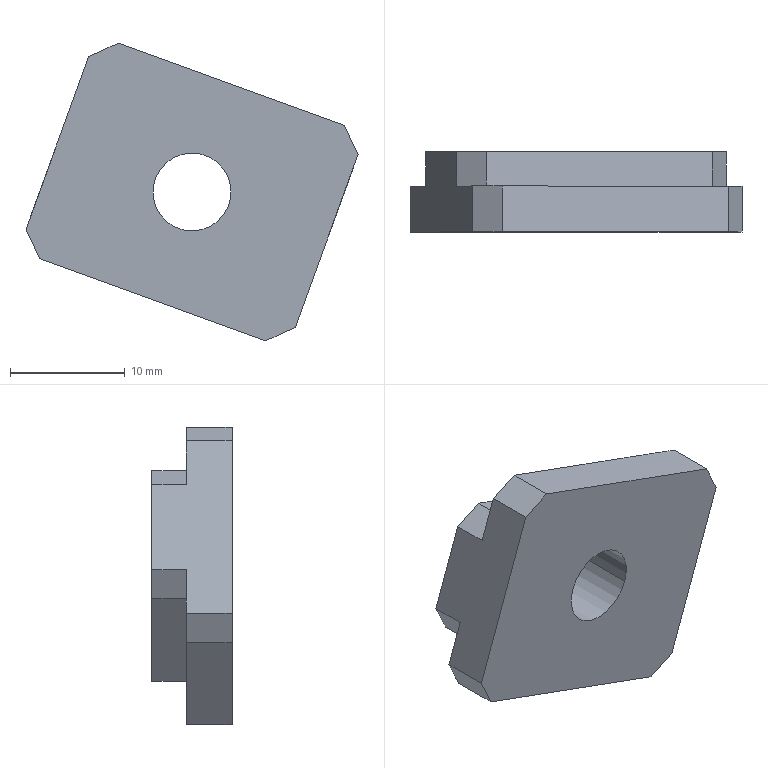Component | SolidWorks | MA060.03.03-07-10 | 1 solid | 20 faces | box 28.96 x 7 x 25.98 mm | volume 2582 mm3 | plane 18 | cylinder 2 | commonest cylinder face diameters 6.8 x2 | material Q235A
build123d program:
from build123d import *

# Parameters (mm, degrees)
SKETCH1_W           = 25
SKETCH1_H           = 20
BOSS_EXTRUDE1_DEPTH = 7
M8_TAPPED_HOLE1_D   = 6.8
SKETCH4_W           = 3
SKETCH4_H           = 4.05
CUT_EXTRUDE1_DEPTH  = 28.821
CHAMFER1_SIZE       = 2


with BuildPart() as part:
    # Sketch1 → Boss-Extrude1 (new body)
    with BuildSketch(Plane.XY):
        Rectangle(SKETCH1_W, SKETCH1_H)
    extrude(amount=BOSS_EXTRUDE1_DEPTH)

    # M8 Tapped Hole1 (through all)
    with Locations(Plane.XY.offset(7)):
        with Locations((0, 0)):
            Hole(M8_TAPPED_HOLE1_D / 2)

    # Sketch4 → Cut-Extrude1 (cut, through all)
    with BuildSketch(Plane(origin=(12.5, 0, 0), x_dir=(0, 0, -1), z_dir=(1, 0, 0))):
        with Locations((-1.5, 7.975)):
            Rectangle(SKETCH4_W, SKETCH4_H)
        with Locations((-1.5, -7.975)):
            Rectangle(SKETCH4_W, SKETCH4_H)
    extrude(amount=-CUT_EXTRUDE1_DEPTH, mode=Mode.SUBTRACT)

    # Chamfer1
    chamfer1_edges = [part.edges().sort_by_distance(p)[0] for p in [
        (-12.5, 5.95, 1.5),
        (12.5, 5.95, 1.5),
        (-12.5, -5.95, 1.5),
        (12.5, -5.95, 1.5),
        (12.5, -10, 5),
        (-12.5, -10, 5),
        (-12.5, 10, 5),
        (12.5, 10, 5),
    ]]
    chamfer(chamfer1_edges, length=CHAMFER1_SIZE)


solid = part.part

# Placed as in the assembly
solid = solid.moved(Location((221.425, 81.053, -80.645), (90, 0, -20)))
STEP:
#1=COLOUR_RGB('',0.7922,0.8196,0.9333);
#2=FILL_AREA_STYLE_COLOUR('',#1);
#3=FILL_AREA_STYLE('',(#2));
#4=SURFACE_STYLE_FILL_AREA(#3);
#5=SURFACE_SIDE_STYLE('',(#4));
#6=SURFACE_STYLE_USAGE(.BOTH.,#5);
#7=PRESENTATION_STYLE_ASSIGNMENT((#6));
#8=CARTESIAN_POINT('',(8.843,3.191,-3.221));
#9=VERTEX_POINT('',#8);
#10=CARTESIAN_POINT('',(8.592,3.191,-3.129));
#11=VERTEX_POINT('',#10);
#12=CARTESIAN_POINT('',(8.718,3.191,-3.175));
#13=DIRECTION('',(-0.,-1.,0.));
#14=DIRECTION('',(-0.9397,0.,0.342));
#15=AXIS2_PLACEMENT_3D('',#12,#13,#14);
#16=CIRCLE('',#15,0.1339);
#17=EDGE_CURVE('',#9,#11,#16,.T.);
#18=ORIENTED_EDGE('',*,*,#17,.F.);
#19=CARTESIAN_POINT('',(8.843,2.915,-3.221));
#20=VERTEX_POINT('',#19);
#21=CARTESIAN_POINT('',(8.843,2.915,-3.221));
#22=DIRECTION('',(-0.,-1.,0.));
#23=VECTOR('',#22,39.37);
#24=LINE('',#21,#23);
#25=EDGE_CURVE('',#9,#20,#24,.T.);
#26=ORIENTED_EDGE('',*,*,#25,.T.);
#27=CARTESIAN_POINT('',(8.592,2.915,-3.129));
#28=VERTEX_POINT('',#27);
#29=CARTESIAN_POINT('',(8.718,2.915,-3.175));
#30=DIRECTION('',(-0.,-1.,0.));
#31=DIRECTION('',(-0.9397,0.,0.342));
#32=AXIS2_PLACEMENT_3D('',#29,#30,#31);
#33=CIRCLE('',#32,0.1339);
#34=EDGE_CURVE('',#20,#28,#33,.T.);
#35=ORIENTED_EDGE('',*,*,#34,.T.);
#36=CARTESIAN_POINT('',(8.592,2.915,-3.129));
#37=DIRECTION('',(-0.,-1.,0.));
#38=VECTOR('',#37,39.37);
#39=LINE('',#36,#38);
#40=EDGE_CURVE('',#11,#28,#39,.T.);
#41=ORIENTED_EDGE('',*,*,#40,.F.);
#42=EDGE_LOOP('',(#18,#26,#35,#41));
#43=FACE_OUTER_BOUND('',#42,.T.);
#44=CARTESIAN_POINT('',(8.718,2.915,-3.175));
#45=DIRECTION('',(-0.,-1.,0.));
#46=DIRECTION('',(-0.9397,0.,0.342));
#47=AXIS2_PLACEMENT_3D('',#44,#45,#46);
#48=CYLINDRICAL_SURFACE('',#47,0.1339);
#49=ADVANCED_FACE('',(#43),#48,.F.);
#50=CARTESIAN_POINT('',(8.308,3.073,-2.861));
#51=VERTEX_POINT('',#50);
#52=CARTESIAN_POINT('',(8.363,3.073,-2.711));
#53=VERTEX_POINT('',#52);
#54=CARTESIAN_POINT('',(8.39,3.073,-2.637));
#55=DIRECTION('',(0.342,-0.,0.9397));
#56=VECTOR('',#55,39.37);
#57=LINE('',#54,#56);
#58=EDGE_CURVE('',#51,#53,#57,.T.);
#59=ORIENTED_EDGE('',*,*,#58,.F.);
#60=CARTESIAN_POINT('',(8.308,3.191,-2.861));
#61=VERTEX_POINT('',#60);
#62=CARTESIAN_POINT('',(8.308,2.915,-2.861));
#63=DIRECTION('',(0.,1.,-0.));
#64=VECTOR('',#63,39.37);
#65=LINE('',#62,#64);
#66=EDGE_CURVE('',#51,#61,#65,.T.);
#67=ORIENTED_EDGE('',*,*,#66,.T.);
#68=CARTESIAN_POINT('',(8.202,3.191,-3.153));
#69=VERTEX_POINT('',#68);
#70=CARTESIAN_POINT('',(8.39,3.191,-2.637));
#71=DIRECTION('',(-0.342,0.,-0.9397));
#72=VECTOR('',#71,39.37);
#73=LINE('',#70,#72);
#74=EDGE_CURVE('',#61,#69,#73,.T.);
#75=ORIENTED_EDGE('',*,*,#74,.T.);
#76=CARTESIAN_POINT('',(8.202,3.073,-3.153));
#77=VERTEX_POINT('',#76);
#78=CARTESIAN_POINT('',(8.202,2.915,-3.153));
#79=DIRECTION('',(-0.,-1.,0.));
#80=VECTOR('',#79,39.37);
#81=LINE('',#78,#80);
#82=EDGE_CURVE('',#69,#77,#81,.T.);
#83=ORIENTED_EDGE('',*,*,#82,.T.);
#84=CARTESIAN_POINT('',(8.147,3.073,-3.303));
#85=VERTEX_POINT('',#84);
#86=CARTESIAN_POINT('',(8.12,3.073,-3.377));
#87=DIRECTION('',(0.342,0.,0.9397));
#88=VECTOR('',#87,39.37);
#89=LINE('',#86,#88);
#90=EDGE_CURVE('',#85,#77,#89,.T.);
#91=ORIENTED_EDGE('',*,*,#90,.F.);
#92=CARTESIAN_POINT('',(8.147,2.915,-3.303));
#93=VERTEX_POINT('',#92);
#94=CARTESIAN_POINT('',(8.147,2.915,-3.303));
#95=DIRECTION('',(-0.,-1.,0.));
#96=VECTOR('',#95,39.37);
#97=LINE('',#94,#96);
#98=EDGE_CURVE('',#85,#93,#97,.T.);
#99=ORIENTED_EDGE('',*,*,#98,.T.);
#100=CARTESIAN_POINT('',(8.363,2.915,-2.711));
#101=VERTEX_POINT('',#100);
#102=CARTESIAN_POINT('',(8.39,2.915,-2.637));
#103=DIRECTION('',(-0.342,0.,-0.9397));
#104=VECTOR('',#103,39.37);
#105=LINE('',#102,#104);
#106=EDGE_CURVE('',#101,#93,#105,.T.);
#107=ORIENTED_EDGE('',*,*,#106,.F.);
#108=CARTESIAN_POINT('',(8.363,2.915,-2.711));
#109=DIRECTION('',(0.,1.,-0.));
#110=VECTOR('',#109,39.37);
#111=LINE('',#108,#110);
#112=EDGE_CURVE('',#101,#53,#111,.T.);
#113=ORIENTED_EDGE('',*,*,#112,.T.);
#114=EDGE_LOOP('',(#59,#67,#75,#83,#91,#99,#107,#113));
#115=FACE_OUTER_BOUND('',#114,.T.);
#116=CARTESIAN_POINT('',(8.39,2.915,-2.637));
#117=DIRECTION('',(0.9397,-0.,-0.342));
#118=DIRECTION('',(-0.,-1.,0.));
#119=AXIS2_PLACEMENT_3D('',#116,#117,#118);
#120=PLANE('',#119);
#121=ADVANCED_FACE('',(#115),#120,.F.);
#122=CARTESIAN_POINT('',(8.194,2.915,-3.404));
#123=VERTEX_POINT('',#122);
#124=CARTESIAN_POINT('',(8.971,2.915,-3.686));
#125=VERTEX_POINT('',#124);
#126=CARTESIAN_POINT('',(9.045,2.915,-3.713));
#127=DIRECTION('',(0.9397,-0.,-0.342));
#128=VECTOR('',#127,39.37);
#129=LINE('',#126,#128);
#130=EDGE_CURVE('',#123,#125,#129,.T.);
#131=ORIENTED_EDGE('',*,*,#130,.F.);
#132=CARTESIAN_POINT('',(8.194,3.073,-3.404));
#133=VERTEX_POINT('',#132);
#134=CARTESIAN_POINT('',(8.194,2.915,-3.404));
#135=DIRECTION('',(0.,1.,-0.));
#136=VECTOR('',#135,39.37);
#137=LINE('',#134,#136);
#138=EDGE_CURVE('',#123,#133,#137,.T.);
#139=ORIENTED_EDGE('',*,*,#138,.T.);
#140=CARTESIAN_POINT('',(8.971,3.073,-3.686));
#141=VERTEX_POINT('',#140);
#142=CARTESIAN_POINT('',(9.045,3.073,-3.713));
#143=DIRECTION('',(-0.9397,0.,0.342));
#144=VECTOR('',#143,39.37);
#145=LINE('',#142,#144);
#146=EDGE_CURVE('',#141,#133,#145,.T.);
#147=ORIENTED_EDGE('',*,*,#146,.F.);
#148=CARTESIAN_POINT('',(8.971,2.915,-3.686));
#149=DIRECTION('',(-0.,-1.,0.));
#150=VECTOR('',#149,39.37);
#151=LINE('',#148,#150);
#152=EDGE_CURVE('',#141,#125,#151,.T.);
#153=ORIENTED_EDGE('',*,*,#152,.T.);
#154=EDGE_LOOP('',(#131,#139,#147,#153));
#155=FACE_OUTER_BOUND('',#154,.T.);
#156=CARTESIAN_POINT('',(9.045,2.915,-3.713));
#157=DIRECTION('',(0.342,-0.,0.9397));
#158=DIRECTION('',(0.,1.,-0.));
#159=AXIS2_PLACEMENT_3D('',#156,#157,#158);
#160=PLANE('',#159);
#161=ADVANCED_FACE('',(#155),#160,.F.);
#162=CARTESIAN_POINT('',(9.233,3.073,-3.197));
#163=VERTEX_POINT('',#162);
#164=CARTESIAN_POINT('',(9.288,3.073,-3.047));
#165=VERTEX_POINT('',#164);
#166=CARTESIAN_POINT('',(9.315,3.073,-2.973));
#167=DIRECTION('',(0.342,-0.,0.9397));
#168=VECTOR('',#167,39.37);
#169=LINE('',#166,#168);
#170=EDGE_CURVE('',#163,#165,#169,.T.);
#171=ORIENTED_EDGE('',*,*,#170,.T.);
#172=CARTESIAN_POINT('',(9.288,2.915,-3.047));
#173=VERTEX_POINT('',#172);
#174=CARTESIAN_POINT('',(9.288,2.915,-3.047));
#175=DIRECTION('',(-0.,-1.,0.));
#176=VECTOR('',#175,39.37);
#177=LINE('',#174,#176);
#178=EDGE_CURVE('',#165,#173,#177,.T.);
#179=ORIENTED_EDGE('',*,*,#178,.T.);
#180=CARTESIAN_POINT('',(9.072,2.915,-3.639));
#181=VERTEX_POINT('',#180);
#182=CARTESIAN_POINT('',(9.315,2.915,-2.973));
#183=DIRECTION('',(0.342,-0.,0.9397));
#184=VECTOR('',#183,39.37);
#185=LINE('',#182,#184);
#186=EDGE_CURVE('',#181,#173,#185,.T.);
#187=ORIENTED_EDGE('',*,*,#186,.F.);
#188=CARTESIAN_POINT('',(9.072,3.073,-3.639));
#189=VERTEX_POINT('',#188);
#190=CARTESIAN_POINT('',(9.072,2.915,-3.639));
#191=DIRECTION('',(0.,1.,-0.));
#192=VECTOR('',#191,39.37);
#193=LINE('',#190,#192);
#194=EDGE_CURVE('',#181,#189,#193,.T.);
#195=ORIENTED_EDGE('',*,*,#194,.T.);
#196=CARTESIAN_POINT('',(9.127,3.073,-3.489));
#197=VERTEX_POINT('',#196);
#198=CARTESIAN_POINT('',(9.045,3.073,-3.713));
#199=DIRECTION('',(0.342,0.,0.9397));
#200=VECTOR('',#199,39.37);
#201=LINE('',#198,#200);
#202=EDGE_CURVE('',#189,#197,#201,.T.);
#203=ORIENTED_EDGE('',*,*,#202,.T.);
#204=CARTESIAN_POINT('',(9.127,3.191,-3.489));
#205=VERTEX_POINT('',#204);
#206=CARTESIAN_POINT('',(9.127,2.915,-3.489));
#207=DIRECTION('',(0.,1.,-0.));
#208=VECTOR('',#207,39.37);
#209=LINE('',#206,#208);
#210=EDGE_CURVE('',#197,#205,#209,.T.);
#211=ORIENTED_EDGE('',*,*,#210,.T.);
#212=CARTESIAN_POINT('',(9.233,3.191,-3.197));
#213=VERTEX_POINT('',#212);
#214=CARTESIAN_POINT('',(9.315,3.191,-2.973));
#215=DIRECTION('',(0.342,-0.,0.9397));
#216=VECTOR('',#215,39.37);
#217=LINE('',#214,#216);
#218=EDGE_CURVE('',#205,#213,#217,.T.);
#219=ORIENTED_EDGE('',*,*,#218,.T.);
#220=CARTESIAN_POINT('',(9.233,2.915,-3.197));
#221=DIRECTION('',(-0.,-1.,0.));
#222=VECTOR('',#221,39.37);
#223=LINE('',#220,#222);
#224=EDGE_CURVE('',#213,#163,#223,.T.);
#225=ORIENTED_EDGE('',*,*,#224,.T.);
#226=EDGE_LOOP('',(#171,#179,#187,#195,#203,#211,#219,#225));
#227=FACE_OUTER_BOUND('',#226,.T.);
#228=CARTESIAN_POINT('',(9.315,2.915,-2.973));
#229=DIRECTION('',(-0.9397,0.,0.342));
#230=DIRECTION('',(0.,1.,-0.));
#231=AXIS2_PLACEMENT_3D('',#228,#229,#230);
#232=PLANE('',#231);
#233=ADVANCED_FACE('',(#227),#232,.F.);
#234=CARTESIAN_POINT('',(9.241,3.073,-2.946));
#235=VERTEX_POINT('',#234);
#236=CARTESIAN_POINT('',(8.464,3.073,-2.664));
#237=VERTEX_POINT('',#236);
#238=CARTESIAN_POINT('',(9.315,3.073,-2.973));
#239=DIRECTION('',(-0.9397,0.,0.342));
#240=VECTOR('',#239,39.37);
#241=LINE('',#238,#240);
#242=EDGE_CURVE('',#235,#237,#241,.T.);
#243=ORIENTED_EDGE('',*,*,#242,.T.);
#244=CARTESIAN_POINT('',(8.464,2.915,-2.664));
#245=VERTEX_POINT('',#244);
#246=CARTESIAN_POINT('',(8.464,2.915,-2.664));
#247=DIRECTION('',(-0.,-1.,0.));
#248=VECTOR('',#247,39.37);
#249=LINE('',#246,#248);
#250=EDGE_CURVE('',#237,#245,#249,.T.);
#251=ORIENTED_EDGE('',*,*,#250,.T.);
#252=CARTESIAN_POINT('',(9.241,2.915,-2.946));
#253=VERTEX_POINT('',#252);
#254=CARTESIAN_POINT('',(9.315,2.915,-2.973));
#255=DIRECTION('',(-0.9397,0.,0.342));
#256=VECTOR('',#255,39.37);
#257=LINE('',#254,#256);
#258=EDGE_CURVE('',#253,#245,#257,.T.);
#259=ORIENTED_EDGE('',*,*,#258,.F.);
#260=CARTESIAN_POINT('',(9.241,2.915,-2.946));
#261=DIRECTION('',(0.,1.,-0.));
#262=VECTOR('',#261,39.37);
#263=LINE('',#260,#262);
#264=EDGE_CURVE('',#253,#235,#263,.T.);
#265=ORIENTED_EDGE('',*,*,#264,.T.);
#266=EDGE_LOOP('',(#243,#251,#259,#265));
#267=FACE_OUTER_BOUND('',#266,.T.);
#268=CARTESIAN_POINT('',(9.315,2.915,-2.973));
#269=DIRECTION('',(-0.342,0.,-0.9397));
#270=DIRECTION('',(-0.,-1.,0.));
#271=AXIS2_PLACEMENT_3D('',#268,#269,#270);
#272=PLANE('',#271);
#273=ADVANCED_FACE('',(#267),#272,.F.);
#274=CARTESIAN_POINT('',(8.718,2.915,-3.175));
#275=DIRECTION('',(-0.,-1.,0.));
#276=DIRECTION('',(-0.9397,0.,0.342));
#277=AXIS2_PLACEMENT_3D('',#274,#275,#276);
#278=CIRCLE('',#277,0.1339);
#279=EDGE_CURVE('',#28,#20,#278,.T.);
#280=ORIENTED_EDGE('',*,*,#279,.F.);
#281=ORIENTED_EDGE('',*,*,#34,.F.);
#282=EDGE_LOOP('',(#280,#281));
#283=FACE_BOUND('',#282,.T.);
#284=ORIENTED_EDGE('',*,*,#106,.T.);
#285=CARTESIAN_POINT('',(8.194,2.915,-3.404));
#286=DIRECTION('',(0.4226,-0.,-0.9063));
#287=VECTOR('',#286,39.37);
#288=LINE('',#285,#287);
#289=EDGE_CURVE('',#93,#123,#288,.T.);
#290=ORIENTED_EDGE('',*,*,#289,.T.);
#291=ORIENTED_EDGE('',*,*,#130,.T.);
#292=CARTESIAN_POINT('',(9.072,2.915,-3.639));
#293=DIRECTION('',(0.9063,-0.,0.4226));
#294=VECTOR('',#293,39.37);
#295=LINE('',#292,#294);
#296=EDGE_CURVE('',#125,#181,#295,.T.);
#297=ORIENTED_EDGE('',*,*,#296,.T.);
#298=ORIENTED_EDGE('',*,*,#186,.T.);
#299=CARTESIAN_POINT('',(9.241,2.915,-2.946));
#300=DIRECTION('',(-0.4226,0.,0.9063));
#301=VECTOR('',#300,39.37);
#302=LINE('',#299,#301);
#303=EDGE_CURVE('',#173,#253,#302,.T.);
#304=ORIENTED_EDGE('',*,*,#303,.T.);
#305=ORIENTED_EDGE('',*,*,#258,.T.);
#306=CARTESIAN_POINT('',(8.363,2.915,-2.711));
#307=DIRECTION('',(-0.9063,0.,-0.4226));
#308=VECTOR('',#307,39.37);
#309=LINE('',#306,#308);
#310=EDGE_CURVE('',#245,#101,#309,.T.);
#311=ORIENTED_EDGE('',*,*,#310,.T.);
#312=EDGE_LOOP('',(#284,#290,#291,#297,#298,#304,#305,#311));
#313=FACE_OUTER_BOUND('',#312,.T.);
#314=CARTESIAN_POINT('',(8.718,2.915,-3.175));
#315=DIRECTION('',(0.,1.,-0.));
#316=DIRECTION('',(0.9397,-0.,-0.342));
#317=AXIS2_PLACEMENT_3D('',#314,#315,#316);
#318=PLANE('',#317);
#319=ADVANCED_FACE('',(#283,#313),#318,.F.);
#320=ORIENTED_EDGE('',*,*,#74,.F.);
#321=CARTESIAN_POINT('',(8.409,3.191,-2.814));
#322=VERTEX_POINT('',#321);
#323=CARTESIAN_POINT('',(8.524,3.191,-2.76));
#324=DIRECTION('',(0.9063,-0.,0.4226));
#325=VECTOR('',#324,39.37);
#326=LINE('',#323,#325);
#327=EDGE_CURVE('',#61,#322,#326,.T.);
#328=ORIENTED_EDGE('',*,*,#327,.T.);
#329=CARTESIAN_POINT('',(9.186,3.191,-3.096));
#330=VERTEX_POINT('',#329);
#331=CARTESIAN_POINT('',(9.26,3.191,-3.123));
#332=DIRECTION('',(-0.9397,0.,0.342));
#333=VECTOR('',#332,39.37);
#334=LINE('',#331,#333);
#335=EDGE_CURVE('',#330,#322,#334,.T.);
#336=ORIENTED_EDGE('',*,*,#335,.F.);
#337=CARTESIAN_POINT('',(9.133,3.191,-2.981));
#338=DIRECTION('',(0.4226,-0.,-0.9063));
#339=VECTOR('',#338,39.37);
#340=LINE('',#337,#339);
#341=EDGE_CURVE('',#330,#213,#340,.T.);
#342=ORIENTED_EDGE('',*,*,#341,.T.);
#343=ORIENTED_EDGE('',*,*,#218,.F.);
#344=CARTESIAN_POINT('',(9.026,3.191,-3.537));
#345=VERTEX_POINT('',#344);
#346=CARTESIAN_POINT('',(8.911,3.191,-3.59));
#347=DIRECTION('',(-0.9063,0.,-0.4226));
#348=VECTOR('',#347,39.37);
#349=LINE('',#346,#348);
#350=EDGE_CURVE('',#205,#345,#349,.T.);
#351=ORIENTED_EDGE('',*,*,#350,.T.);
#352=CARTESIAN_POINT('',(8.249,3.191,-3.254));
#353=VERTEX_POINT('',#352);
#354=CARTESIAN_POINT('',(9.1,3.191,-3.563));
#355=DIRECTION('',(-0.9397,0.,0.342));
#356=VECTOR('',#355,39.37);
#357=LINE('',#354,#356);
#358=EDGE_CURVE('',#345,#353,#357,.T.);
#359=ORIENTED_EDGE('',*,*,#358,.T.);
#360=CARTESIAN_POINT('',(8.302,3.191,-3.369));
#361=DIRECTION('',(-0.4226,0.,0.9063));
#362=VECTOR('',#361,39.37);
#363=LINE('',#360,#362);
#364=EDGE_CURVE('',#353,#69,#363,.T.);
#365=ORIENTED_EDGE('',*,*,#364,.T.);
#366=EDGE_LOOP('',(#320,#328,#336,#342,#343,#351,#359,#365));
#367=FACE_OUTER_BOUND('',#366,.T.);
#368=CARTESIAN_POINT('',(8.718,3.191,-3.175));
#369=DIRECTION('',(-0.,-1.,0.));
#370=DIRECTION('',(-0.9397,0.,0.342));
#371=AXIS2_PLACEMENT_3D('',#368,#369,#370);
#372=CIRCLE('',#371,0.1339);
#373=EDGE_CURVE('',#11,#9,#372,.T.);
#374=ORIENTED_EDGE('',*,*,#373,.T.);
#375=ORIENTED_EDGE('',*,*,#17,.T.);
#376=EDGE_LOOP('',(#374,#375));
#377=FACE_BOUND('',#376,.T.);
#378=CARTESIAN_POINT('',(8.718,3.191,-3.175));
#379=DIRECTION('',(0.,1.,-0.));
#380=DIRECTION('',(0.9397,-0.,-0.342));
#381=AXIS2_PLACEMENT_3D('',#378,#379,#380);
#382=PLANE('',#381);
#383=ADVANCED_FACE('',(#367,#377),#382,.T.);
#384=ORIENTED_EDGE('',*,*,#25,.F.);
#385=ORIENTED_EDGE('',*,*,#373,.F.);
#386=ORIENTED_EDGE('',*,*,#40,.T.);
#387=ORIENTED_EDGE('',*,*,#279,.T.);
#388=EDGE_LOOP('',(#384,#385,#386,#387));
#389=FACE_OUTER_BOUND('',#388,.T.);
#390=CARTESIAN_POINT('',(8.718,2.915,-3.175));
#391=DIRECTION('',(-0.,-1.,0.));
#392=DIRECTION('',(-0.9397,0.,0.342));
#393=AXIS2_PLACEMENT_3D('',#390,#391,#392);
#394=CYLINDRICAL_SURFACE('',#393,0.1339);
#395=ADVANCED_FACE('',(#389),#394,.F.);
#396=CARTESIAN_POINT('',(9.026,3.073,-3.537));
#397=VERTEX_POINT('',#396);
#398=CARTESIAN_POINT('',(8.249,3.073,-3.254));
#399=VERTEX_POINT('',#398);
#400=CARTESIAN_POINT('',(9.1,3.073,-3.563));
#401=DIRECTION('',(-0.9397,0.,0.342));
#402=VECTOR('',#401,39.37);
#403=LINE('',#400,#402);
#404=EDGE_CURVE('',#397,#399,#403,.T.);
#405=ORIENTED_EDGE('',*,*,#404,.T.);
#406=CARTESIAN_POINT('',(8.249,3.191,-3.254));
#407=DIRECTION('',(0.,1.,-0.));
#408=VECTOR('',#407,39.37);
#409=LINE('',#406,#408);
#410=EDGE_CURVE('',#399,#353,#409,.T.);
#411=ORIENTED_EDGE('',*,*,#410,.T.);
#412=ORIENTED_EDGE('',*,*,#358,.F.);
#413=CARTESIAN_POINT('',(9.026,3.191,-3.537));
#414=DIRECTION('',(-0.,-1.,0.));
#415=VECTOR('',#414,39.37);
#416=LINE('',#413,#415);
#417=EDGE_CURVE('',#345,#397,#416,.T.);
#418=ORIENTED_EDGE('',*,*,#417,.T.);
#419=EDGE_LOOP('',(#405,#411,#412,#418));
#420=FACE_OUTER_BOUND('',#419,.T.);
#421=CARTESIAN_POINT('',(9.1,3.191,-3.563));
#422=DIRECTION('',(0.342,-0.,0.9397));
#423=DIRECTION('',(0.,1.,-0.));
#424=AXIS2_PLACEMENT_3D('',#421,#422,#423);
#425=PLANE('',#424);
#426=ADVANCED_FACE('',(#420),#425,.F.);
#427=ORIENTED_EDGE('',*,*,#146,.T.);
#428=CARTESIAN_POINT('',(8.194,3.073,-3.404));
#429=DIRECTION('',(-0.4226,0.,0.9063));
#430=VECTOR('',#429,39.37);
#431=LINE('',#428,#430);
#432=EDGE_CURVE('',#133,#85,#431,.T.);
#433=ORIENTED_EDGE('',*,*,#432,.T.);
#434=ORIENTED_EDGE('',*,*,#90,.T.);
#435=CARTESIAN_POINT('',(8.567,3.073,-3.936));
#436=DIRECTION('',(0.4226,-0.,-0.9063));
#437=VECTOR('',#436,39.37);
#438=LINE('',#435,#437);
#439=EDGE_CURVE('',#77,#399,#438,.T.);
#440=ORIENTED_EDGE('',*,*,#439,.T.);
#441=ORIENTED_EDGE('',*,*,#404,.F.);
#442=CARTESIAN_POINT('',(8.974,3.073,-3.561));
#443=DIRECTION('',(0.9063,0.,0.4226));
#444=VECTOR('',#443,39.37);
#445=LINE('',#442,#444);
#446=EDGE_CURVE('',#397,#197,#445,.T.);
#447=ORIENTED_EDGE('',*,*,#446,.T.);
#448=ORIENTED_EDGE('',*,*,#202,.F.);
#449=CARTESIAN_POINT('',(9.072,3.073,-3.639));
#450=DIRECTION('',(-0.9063,-0.,-0.4226));
#451=VECTOR('',#450,39.37);
#452=LINE('',#449,#451);
#453=EDGE_CURVE('',#189,#141,#452,.T.);
#454=ORIENTED_EDGE('',*,*,#453,.T.);
#455=EDGE_LOOP('',(#427,#433,#434,#440,#441,#447,#448,#454));
#456=FACE_OUTER_BOUND('',#455,.T.);
#457=CARTESIAN_POINT('',(9.045,3.073,-3.713));
#458=DIRECTION('',(-0.,-1.,0.));
#459=DIRECTION('',(0.342,0.,0.9397));
#460=AXIS2_PLACEMENT_3D('',#457,#458,#459);
#461=PLANE('',#460);
#462=ADVANCED_FACE('',(#456),#461,.F.);
#463=ORIENTED_EDGE('',*,*,#58,.T.);
#464=CARTESIAN_POINT('',(8.363,3.073,-2.711));
#465=DIRECTION('',(0.9063,-0.,0.4226));
#466=VECTOR('',#465,39.37);
#467=LINE('',#464,#466);
#468=EDGE_CURVE('',#53,#237,#467,.T.);
#469=ORIENTED_EDGE('',*,*,#468,.T.);
#470=ORIENTED_EDGE('',*,*,#242,.F.);
#471=CARTESIAN_POINT('',(9.241,3.073,-2.946));
#472=DIRECTION('',(0.4226,0.,-0.9063));
#473=VECTOR('',#472,39.37);
#474=LINE('',#471,#473);
#475=EDGE_CURVE('',#235,#165,#474,.T.);
#476=ORIENTED_EDGE('',*,*,#475,.T.);
#477=ORIENTED_EDGE('',*,*,#170,.F.);
#478=CARTESIAN_POINT('',(9.186,3.073,-3.096));
#479=VERTEX_POINT('',#478);
#480=CARTESIAN_POINT('',(9.162,3.073,-3.045));
#481=DIRECTION('',(-0.4226,-0.,0.9063));
#482=VECTOR('',#481,39.37);
#483=LINE('',#480,#482);
#484=EDGE_CURVE('',#163,#479,#483,.T.);
#485=ORIENTED_EDGE('',*,*,#484,.T.);
#486=CARTESIAN_POINT('',(8.409,3.073,-2.814));
#487=VERTEX_POINT('',#486);
#488=CARTESIAN_POINT('',(9.26,3.073,-3.123));
#489=DIRECTION('',(-0.9397,0.,0.342));
#490=VECTOR('',#489,39.37);
#491=LINE('',#488,#490);
#492=EDGE_CURVE('',#479,#487,#491,.T.);
#493=ORIENTED_EDGE('',*,*,#492,.T.);
#494=CARTESIAN_POINT('',(9.092,3.073,-2.495));
#495=DIRECTION('',(-0.9063,0.,-0.4226));
#496=VECTOR('',#495,39.37);
#497=LINE('',#494,#496);
#498=EDGE_CURVE('',#487,#51,#497,.T.);
#499=ORIENTED_EDGE('',*,*,#498,.T.);
#500=EDGE_LOOP('',(#463,#469,#470,#476,#477,#485,#493,#499));
#501=FACE_OUTER_BOUND('',#500,.T.);
#502=CARTESIAN_POINT('',(9.315,3.073,-2.973));
#503=DIRECTION('',(-0.,-1.,-0.));
#504=DIRECTION('',(0.342,-0.,0.9397));
#505=AXIS2_PLACEMENT_3D('',#502,#503,#504);
#506=PLANE('',#505);
#507=ADVANCED_FACE('',(#501),#506,.F.);
#508=ORIENTED_EDGE('',*,*,#335,.T.);
#509=CARTESIAN_POINT('',(8.409,3.191,-2.814));
#510=DIRECTION('',(-0.,-1.,0.));
#511=VECTOR('',#510,39.37);
#512=LINE('',#509,#511);
#513=EDGE_CURVE('',#322,#487,#512,.T.);
#514=ORIENTED_EDGE('',*,*,#513,.T.);
#515=ORIENTED_EDGE('',*,*,#492,.F.);
#516=CARTESIAN_POINT('',(9.186,3.191,-3.096));
#517=DIRECTION('',(0.,1.,-0.));
#518=VECTOR('',#517,39.37);
#519=LINE('',#516,#518);
#520=EDGE_CURVE('',#479,#330,#519,.T.);
#521=ORIENTED_EDGE('',*,*,#520,.T.);
#522=EDGE_LOOP('',(#508,#514,#515,#521));
#523=FACE_OUTER_BOUND('',#522,.T.);
#524=CARTESIAN_POINT('',(9.26,3.191,-3.123));
#525=DIRECTION('',(-0.342,0.,-0.9397));
#526=DIRECTION('',(-0.,-1.,0.));
#527=AXIS2_PLACEMENT_3D('',#524,#525,#526);
#528=PLANE('',#527);
#529=ADVANCED_FACE('',(#523),#528,.F.);
#530=ORIENTED_EDGE('',*,*,#327,.F.);
#531=ORIENTED_EDGE('',*,*,#66,.F.);
#532=ORIENTED_EDGE('',*,*,#498,.F.);
#533=ORIENTED_EDGE('',*,*,#513,.F.);
#534=EDGE_LOOP('',(#530,#531,#532,#533));
#535=FACE_OUTER_BOUND('',#534,.T.);
#536=CARTESIAN_POINT('',(8.409,3.191,-2.814));
#537=DIRECTION('',(0.4226,-0.,-0.9063));
#538=DIRECTION('',(-0.,-1.,0.));
#539=AXIS2_PLACEMENT_3D('',#536,#537,#538);
#540=PLANE('',#539);
#541=ADVANCED_FACE('',(#535),#540,.F.);
#542=ORIENTED_EDGE('',*,*,#439,.F.);
#543=ORIENTED_EDGE('',*,*,#82,.F.);
#544=ORIENTED_EDGE('',*,*,#364,.F.);
#545=ORIENTED_EDGE('',*,*,#410,.F.);
#546=EDGE_LOOP('',(#542,#543,#544,#545));
#547=FACE_OUTER_BOUND('',#546,.T.);
#548=CARTESIAN_POINT('',(8.249,3.191,-3.254));
#549=DIRECTION('',(0.9063,-0.,0.4226));
#550=DIRECTION('',(0.,1.,-0.));
#551=AXIS2_PLACEMENT_3D('',#548,#549,#550);
#552=PLANE('',#551);
#553=ADVANCED_FACE('',(#547),#552,.F.);
#554=ORIENTED_EDGE('',*,*,#289,.F.);
#555=ORIENTED_EDGE('',*,*,#98,.F.);
#556=ORIENTED_EDGE('',*,*,#432,.F.);
#557=ORIENTED_EDGE('',*,*,#138,.F.);
#558=EDGE_LOOP('',(#554,#555,#556,#557));
#559=FACE_OUTER_BOUND('',#558,.T.);
#560=CARTESIAN_POINT('',(8.194,2.915,-3.404));
#561=DIRECTION('',(0.9063,-0.,0.4226));
#562=DIRECTION('',(0.,1.,-0.));
#563=AXIS2_PLACEMENT_3D('',#560,#561,#562);
#564=PLANE('',#563);
#565=ADVANCED_FACE('',(#559),#564,.F.);
#566=ORIENTED_EDGE('',*,*,#310,.F.);
#567=ORIENTED_EDGE('',*,*,#250,.F.);
#568=ORIENTED_EDGE('',*,*,#468,.F.);
#569=ORIENTED_EDGE('',*,*,#112,.F.);
#570=EDGE_LOOP('',(#566,#567,#568,#569));
#571=FACE_OUTER_BOUND('',#570,.T.);
#572=CARTESIAN_POINT('',(8.363,2.915,-2.711));
#573=DIRECTION('',(0.4226,-0.,-0.9063));
#574=DIRECTION('',(0.,1.,-0.));
#575=AXIS2_PLACEMENT_3D('',#572,#573,#574);
#576=PLANE('',#575);
#577=ADVANCED_FACE('',(#571),#576,.F.);
#578=ORIENTED_EDGE('',*,*,#303,.F.);
#579=ORIENTED_EDGE('',*,*,#178,.F.);
#580=ORIENTED_EDGE('',*,*,#475,.F.);
#581=ORIENTED_EDGE('',*,*,#264,.F.);
#582=EDGE_LOOP('',(#578,#579,#580,#581));
#583=FACE_OUTER_BOUND('',#582,.T.);
#584=CARTESIAN_POINT('',(9.241,2.915,-2.946));
#585=DIRECTION('',(-0.9063,0.,-0.4226));
#586=DIRECTION('',(0.,1.,-0.));
#587=AXIS2_PLACEMENT_3D('',#584,#585,#586);
#588=PLANE('',#587);
#589=ADVANCED_FACE('',(#583),#588,.F.);
#590=ORIENTED_EDGE('',*,*,#341,.F.);
#591=ORIENTED_EDGE('',*,*,#520,.F.);
#592=ORIENTED_EDGE('',*,*,#484,.F.);
#593=ORIENTED_EDGE('',*,*,#224,.F.);
#594=EDGE_LOOP('',(#590,#591,#592,#593));
#595=FACE_OUTER_BOUND('',#594,.T.);
#596=CARTESIAN_POINT('',(9.233,2.915,-3.197));
#597=DIRECTION('',(-0.9063,0.,-0.4226));
#598=DIRECTION('',(-0.,-1.,0.));
#599=AXIS2_PLACEMENT_3D('',#596,#597,#598);
#600=PLANE('',#599);
#601=ADVANCED_FACE('',(#595),#600,.F.);
#602=ORIENTED_EDGE('',*,*,#446,.F.);
#603=ORIENTED_EDGE('',*,*,#417,.F.);
#604=ORIENTED_EDGE('',*,*,#350,.F.);
#605=ORIENTED_EDGE('',*,*,#210,.F.);
#606=EDGE_LOOP('',(#602,#603,#604,#605));
#607=FACE_OUTER_BOUND('',#606,.T.);
#608=CARTESIAN_POINT('',(9.127,2.915,-3.489));
#609=DIRECTION('',(-0.4226,0.,0.9063));
#610=DIRECTION('',(0.,1.,-0.));
#611=AXIS2_PLACEMENT_3D('',#608,#609,#610);
#612=PLANE('',#611);
#613=ADVANCED_FACE('',(#607),#612,.F.);
#614=ORIENTED_EDGE('',*,*,#296,.F.);
#615=ORIENTED_EDGE('',*,*,#152,.F.);
#616=ORIENTED_EDGE('',*,*,#453,.F.);
#617=ORIENTED_EDGE('',*,*,#194,.F.);
#618=EDGE_LOOP('',(#614,#615,#616,#617));
#619=FACE_OUTER_BOUND('',#618,.T.);
#620=CARTESIAN_POINT('',(9.072,2.915,-3.639));
#621=DIRECTION('',(-0.4226,0.,0.9063));
#622=DIRECTION('',(0.,1.,-0.));
#623=AXIS2_PLACEMENT_3D('',#620,#621,#622);
#624=PLANE('',#623);
#625=ADVANCED_FACE('',(#619),#624,.F.);
#626=CLOSED_SHELL('',(#49,#121,#161,#233,#273,#319,#383,#395,#426,#462,#507,#529,#541,#553,#565,#577,#589,#601,#613,#625));
#627=MANIFOLD_SOLID_BREP('',#626);
#628=STYLED_ITEM('',(#7),#627);
#629=PRESENTATION_LAYER_ASSIGNMENT('','',(#628));
#630=(LENGTH_UNIT()NAMED_UNIT(*)SI_UNIT($,.METRE.));
#631=LENGTH_MEASURE_WITH_UNIT(LENGTH_MEASURE(0.0254),#630);
#632=DIMENSIONAL_EXPONENTS(1.,0.,0.,0.,0.,0.,0.);
#633=(CONVERSION_BASED_UNIT('',#631)LENGTH_UNIT()NAMED_UNIT(#632));
#634=UNCERTAINTY_MEASURE_WITH_UNIT(LENGTH_MEASURE(0.00001),#633,'','');
#635=(NAMED_UNIT(*)PLANE_ANGLE_UNIT()SI_UNIT($,.RADIAN.));
#636=(NAMED_UNIT(*)SI_UNIT($,.STERADIAN.)SOLID_ANGLE_UNIT());
#637=(GEOMETRIC_REPRESENTATION_CONTEXT(3)GLOBAL_UNCERTAINTY_ASSIGNED_CONTEXT((#634))GLOBAL_UNIT_ASSIGNED_CONTEXT((#633,#635,#636))REPRESENTATION_CONTEXT('',''));
#638=MECHANICAL_DESIGN_GEOMETRIC_PRESENTATION_REPRESENTATION('',(#628),#637);
#639=CARTESIAN_POINT('',(0.,0.,0.));
#640=DIRECTION('',(0.,0.,1.));
#641=DIRECTION('',(1.,0.,0.));
#642=AXIS2_PLACEMENT_3D('',#639,#640,#641);
#643=(LENGTH_UNIT()NAMED_UNIT(*)SI_UNIT($,.METRE.));
#644=LENGTH_MEASURE_WITH_UNIT(LENGTH_MEASURE(0.0254),#643);
#645=DIMENSIONAL_EXPONENTS(1.,0.,0.,0.,0.,0.,0.);
#646=(CONVERSION_BASED_UNIT('',#644)LENGTH_UNIT()NAMED_UNIT(#645));
#647=UNCERTAINTY_MEASURE_WITH_UNIT(LENGTH_MEASURE(0.00001),#646,'','');
#648=(NAMED_UNIT(*)PLANE_ANGLE_UNIT()SI_UNIT($,.RADIAN.));
#649=(NAMED_UNIT(*)SI_UNIT($,.STERADIAN.)SOLID_ANGLE_UNIT());
#650=(GEOMETRIC_REPRESENTATION_CONTEXT(3)GLOBAL_UNCERTAINTY_ASSIGNED_CONTEXT((#647))GLOBAL_UNIT_ASSIGNED_CONTEXT((#646,#648,#649))REPRESENTATION_CONTEXT('',''));
#651=ADVANCED_BREP_SHAPE_REPRESENTATION('',(#627,#642),#650);